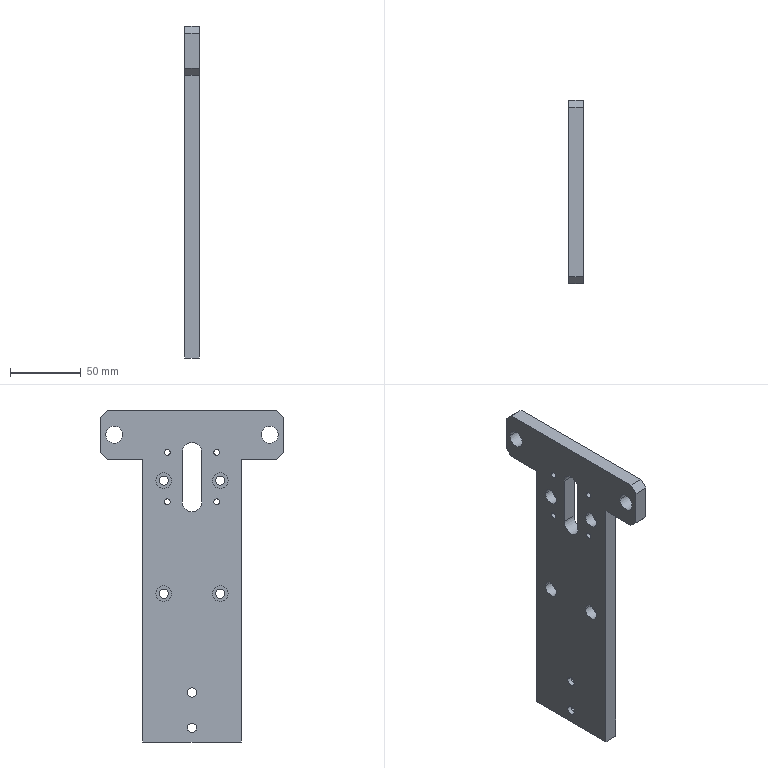Component | SolidWorks | 01-07MarkingMachineDrumConnectingPlate1-1 | 1 solid | 60 faces | box 10 x 130 x 235 mm | volume 171210 mm3 | cylinder 38 | plane 22 | commonest cylinder face diameters 11 x12 6.6 x12 4.2 x8 12 x4 14 x2 | material A3 Steel
build123d program:
from build123d import *

# Parameters (mm, degrees)
BOSS_EXTRUDE1_DEPTH                                = 5
CHAMFER1_SIZE                                      = 5
CUT_EXTRUDE1_DEPTH                                 = 245.029
CUT_EXTRUDE1_DEPTH_BACK                            = 245.029
SKETCH2_R                                          = 6
HOLE_SIZE_ACCORDING_TO_TYPE_1_OF_HEXAG_D           = 6.6
HOLE_SIZE_ACCORDING_TO_TYPE_1_OF_HEXAG_CBORE_D     = 11
HOLE_SIZE_ACCORDING_TO_TYPE_1_OF_HEXAG_CBORE_DEPTH = 6.8
HOLE_SIZE_ACCORDING_TO_TYPE_2_OF_HEXAG_D           = 6.6
HOLE_SIZE_ACCORDING_TO_TYPE_2_OF_HEXAG_CBORE_D     = 11
HOLE_SIZE_ACCORDING_TO_TYPE_2_OF_HEXAG_CBORE_DEPTH = 6.8
M5_TAPPED_HOLE1_D                                  = 4.2
CUT_EXTRUDE2_DEPTH                                 = 245.029


with BuildPart() as part:
    # Sketch1 → Boss-Extrude1 (new, symmetric)
    with BuildSketch(Plane.XY):
        Polygon((65, 0), (-65, 0), (-65, 35), (-35, 35), (-35, 235), (35, 235), (35, 35), (65, 35), align=None)
    extrude(amount=BOSS_EXTRUDE1_DEPTH, both=True)

    # Chamfer1
    chamfer1_edges = [part.edges().sort_by_distance(p)[0] for p in [
        (-65, 35, 0),
        (65, 35, 0),
        (65, 0, 0),
        (-65, 0, 0),
    ]]
    chamfer(chamfer1_edges, length=CHAMFER1_SIZE)

    # Sketch2 → Cut-Extrude1 (cut, two sides: drawn at the far end of the back side and taken through both)
    with BuildSketch(Plane.XY.offset(5).offset(-CUT_EXTRUDE1_DEPTH_BACK)):
        with Locations((-55, 17.5)):
            Circle(SKETCH2_R)
        with Locations(Location((55, 17.5, 0), (0, 0, 180))):
            Circle(SKETCH2_R)
    extrude(amount=CUT_EXTRUDE1_DEPTH + CUT_EXTRUDE1_DEPTH_BACK, mode=Mode.SUBTRACT)

    # Hole Size _According to_ Type 1 of Hexag (through all)
    with Locations(Plane(origin=(-20, 50, 5), x_dir=(1, 0, 0), z_dir=(0, 0, 1))):
        with Locations((0, 0), (0, 80), (40, 80), (40, 0)):
            CounterBoreHole(HOLE_SIZE_ACCORDING_TO_TYPE_1_OF_HEXAG_D / 2, HOLE_SIZE_ACCORDING_TO_TYPE_1_OF_HEXAG_CBORE_D / 2, HOLE_SIZE_ACCORDING_TO_TYPE_1_OF_HEXAG_CBORE_DEPTH)

    # Hole Size _According to_ Type 2 of Hexag (through all)
    with Locations(Plane(origin=(0, 225, -5), x_dir=(-1, 0, 0), z_dir=(0, 0, -1))):
        with Locations((0, 0), (0, -25)):
            CounterBoreHole(HOLE_SIZE_ACCORDING_TO_TYPE_2_OF_HEXAG_D / 2, HOLE_SIZE_ACCORDING_TO_TYPE_2_OF_HEXAG_CBORE_D / 2, HOLE_SIZE_ACCORDING_TO_TYPE_2_OF_HEXAG_CBORE_DEPTH)

    # M5 Tapped Hole1 (through all)
    with Locations(Plane(origin=(-17.5, 65, -5), x_dir=(-1, 0, 0), z_dir=(0, 0, -1))):
        with Locations((0, 0), (0, -35), (-35, -35), (-35, 0)):
            Hole(M5_TAPPED_HOLE1_D / 2)

    # Sketch11 → Cut-Extrude2 (cut, through all)
    with BuildSketch(Plane.XY.offset(5)):
        with BuildLine():
            Line((-7, 30), (-7, 65))
            ThreePointArc((-7, 65), (0, 72), (7, 65))
            Line((7, 65), (7, 30))
            ThreePointArc((7, 30), (0, 23), (-7, 30))
        make_face()
    extrude(amount=-CUT_EXTRUDE2_DEPTH, mode=Mode.SUBTRACT)


solid = part.part

# Placed as in the assembly
solid = solid.moved(Location((-61.91, 2.41, 45), (-90, -90, 0)))